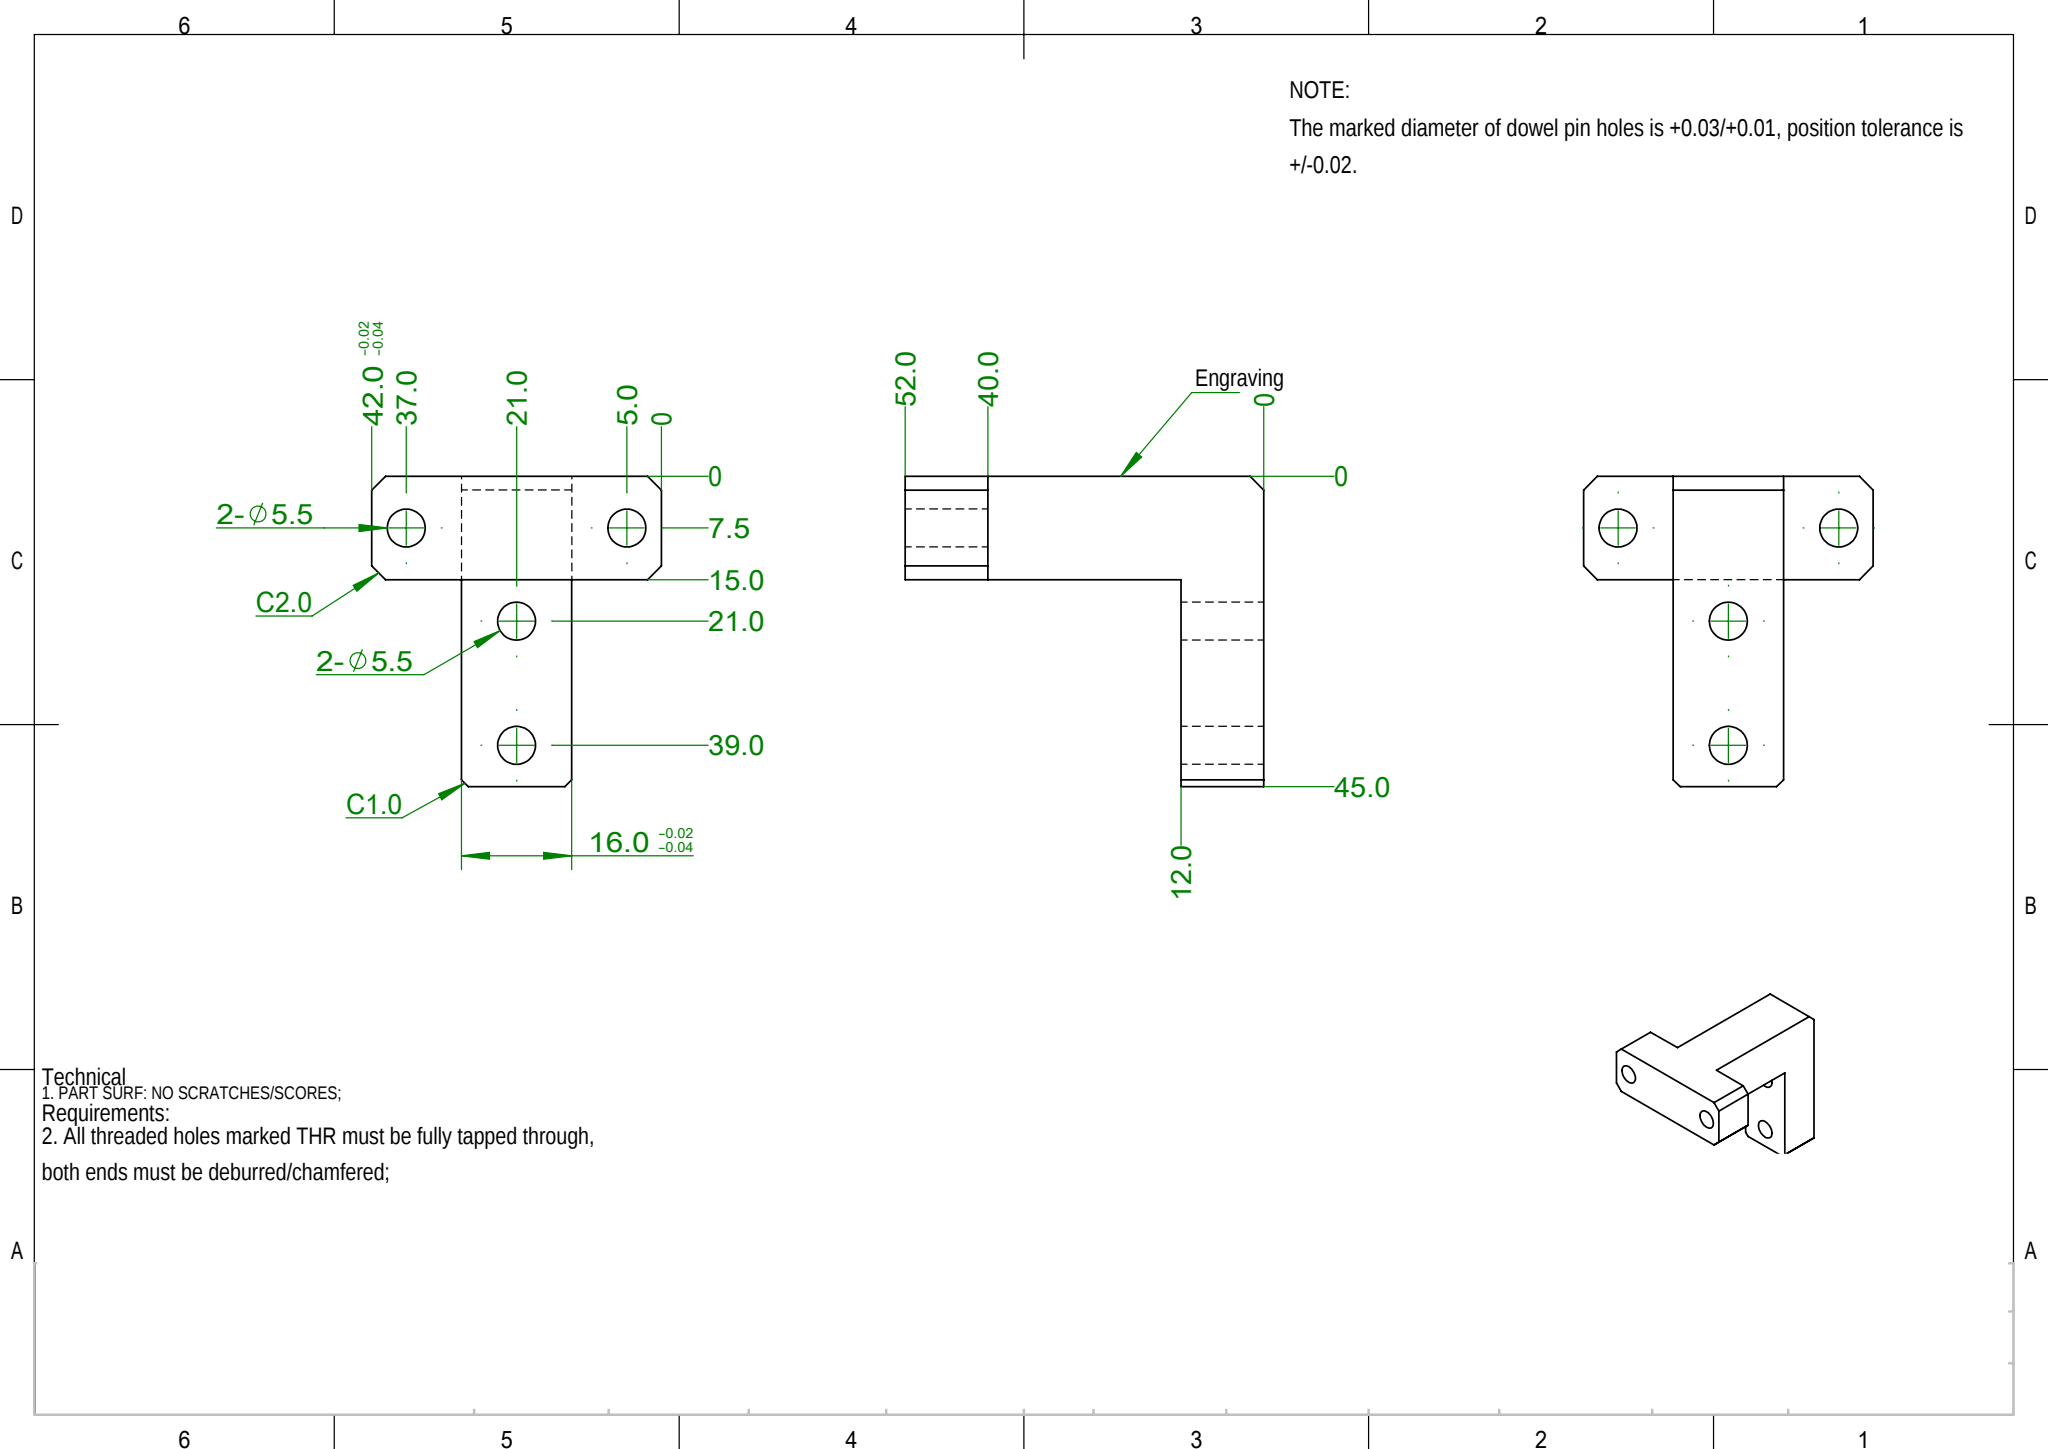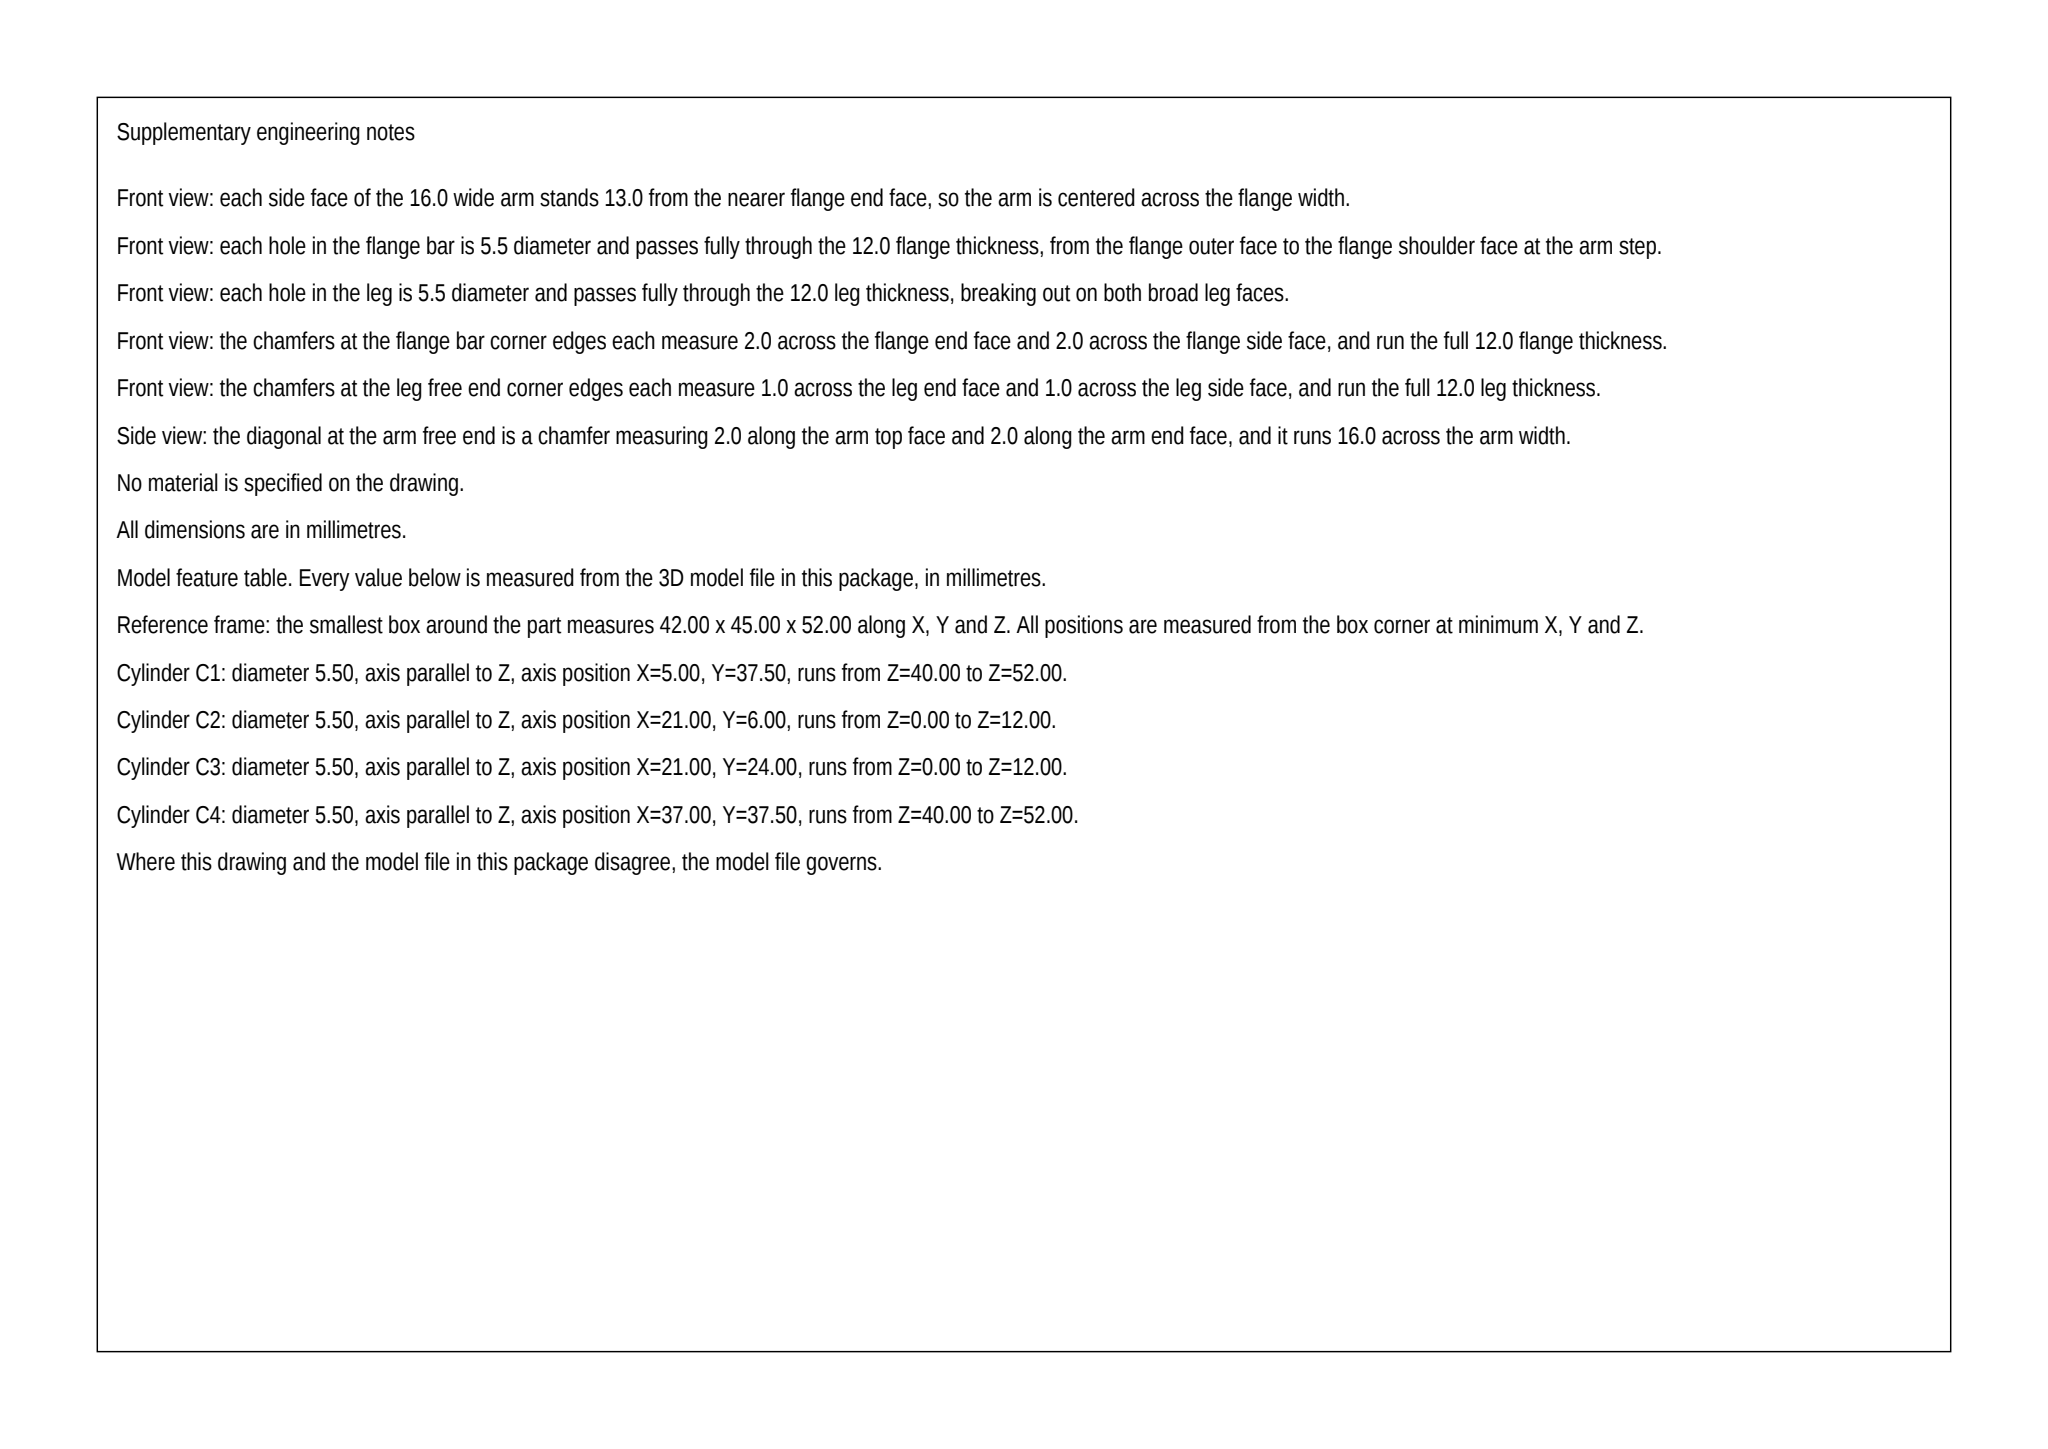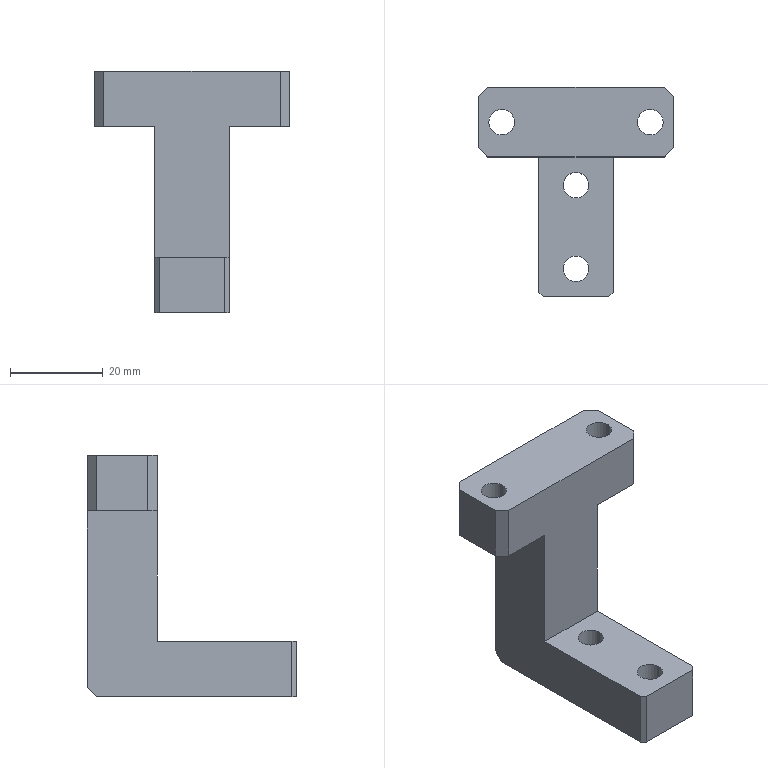Part | SolidWorks | mm | 1 solid | 27 faces | box 42 x 45 x 52 mm | volume 21640 mm3 | plane 19 | cylinder 8 | commonest cylinder face diameters 5.5 x8
Drawing notes:
ALL DIMENSIONS ARE IN MILLIMETERS (mm). | from the solid: STEP model units are mm (bbox_xyz 42.0 x 45.0 x 52.0 mm)
4X PIN HOLE Ø5.5 +0.03/+0.01, TRUE POS ±0.02, THRU 12 | from the solid: cylinders dia 5.5 axis z length 12 at (5.0,37.5),(37.0,37.5),(21.0,24.0),(21.0,6.0); plate thk z 0-12
OVERALL WIDTH 42.0 MM IN X, MEASURED FROM LEFT END FACE (X=0 DATUM) TO RIGHT END FACE. | from the solid: bbox_xyz = [42.0, 45.0, 52.0]; axis_planes x=0.0 and x=42.0
RIGHT-HAND Ø5.5 THRU HOLE (12 DEEP): AXIS AT X=37.0 FROM LEFT END FACE, Y=7.5 FROM TOP FACE (37.5 FROM BOTTOM Y=0 DATUM). | from the solid: cylinders [5.5, z, [37.0, 37.5], 12.0]; bbox Y=45.0
PIN HOLES: 4X Ø5.5 THRU 12 AT X=5.0 AND X=37.0 (Y=37.5 FROM Y=0 DATUM) AND X=21.0 (Y=24.0 AND Y=6.0 FROM Y=0 DATUM). | from the solid: cylinders [5.5,z,[5.0,37.5],12.0], [5.5,z,[37.0,37.5],12.0], [5.5,z,[21.0,24.0],12.0], [5.5,z,[21.0,6.0],12.0]
STEP:
#1=CARTESIAN_POINT('',(-2.75,-13.5,12.));
#2=VERTEX_POINT('',#1);
#3=CARTESIAN_POINT('',(2.75,-13.5,12.));
#4=VERTEX_POINT('',#3);
#5=CARTESIAN_POINT('',(-0.,-13.5,12.));
#6=DIRECTION('',(0.,0.,1.));
#7=DIRECTION('',(1.,0.,0.));
#8=AXIS2_PLACEMENT_3D('',#5,#6,#7);
#9=CIRCLE('',#8,2.75);
#10=EDGE_CURVE('',#2,#4,#9,.T.);
#11=ORIENTED_EDGE('',*,*,#10,.F.);
#12=CARTESIAN_POINT('',(-2.75,-13.5,24.));
#13=VERTEX_POINT('',#12);
#14=CARTESIAN_POINT('',(-2.75,-13.5,-87.));
#15=DIRECTION('',(0.,0.,1.));
#16=VECTOR('',#15,1000.);
#17=LINE('',#14,#16);
#18=EDGE_CURVE('',#2,#13,#17,.T.);
#19=ORIENTED_EDGE('',*,*,#18,.T.);
#20=CARTESIAN_POINT('',(2.75,-13.5,24.));
#21=VERTEX_POINT('',#20);
#22=CARTESIAN_POINT('',(-0.,-13.5,24.));
#23=DIRECTION('',(0.,0.,1.));
#24=DIRECTION('',(1.,0.,0.));
#25=AXIS2_PLACEMENT_3D('',#22,#23,#24);
#26=CIRCLE('',#25,2.75);
#27=EDGE_CURVE('',#13,#21,#26,.T.);
#28=ORIENTED_EDGE('',*,*,#27,.T.);
#29=CARTESIAN_POINT('',(2.75,-13.5,-87.));
#30=DIRECTION('',(0.,0.,1.));
#31=VECTOR('',#30,1000.);
#32=LINE('',#29,#31);
#33=EDGE_CURVE('',#4,#21,#32,.T.);
#34=ORIENTED_EDGE('',*,*,#33,.F.);
#35=EDGE_LOOP('',(#11,#19,#28,#34));
#36=FACE_OUTER_BOUND('',#35,.T.);
#37=CARTESIAN_POINT('',(-0.,-13.5,-87.));
#38=DIRECTION('',(0.,0.,1.));
#39=DIRECTION('',(1.,0.,0.));
#40=AXIS2_PLACEMENT_3D('',#37,#38,#39);
#41=CYLINDRICAL_SURFACE('',#40,2.75);
#42=ADVANCED_FACE('',(#36),#41,.F.);
#43=CARTESIAN_POINT('',(-2.75,-31.5,12.));
#44=VERTEX_POINT('',#43);
#45=CARTESIAN_POINT('',(2.75,-31.5,12.));
#46=VERTEX_POINT('',#45);
#47=CARTESIAN_POINT('',(-0.,-31.5,12.));
#48=DIRECTION('',(0.,0.,1.));
#49=DIRECTION('',(1.,0.,0.));
#50=AXIS2_PLACEMENT_3D('',#47,#48,#49);
#51=CIRCLE('',#50,2.75);
#52=EDGE_CURVE('',#44,#46,#51,.T.);
#53=ORIENTED_EDGE('',*,*,#52,.F.);
#54=CARTESIAN_POINT('',(-2.75,-31.5,24.));
#55=VERTEX_POINT('',#54);
#56=CARTESIAN_POINT('',(-2.75,-31.5,-87.));
#57=DIRECTION('',(0.,0.,1.));
#58=VECTOR('',#57,1000.);
#59=LINE('',#56,#58);
#60=EDGE_CURVE('',#44,#55,#59,.T.);
#61=ORIENTED_EDGE('',*,*,#60,.T.);
#62=CARTESIAN_POINT('',(2.75,-31.5,24.));
#63=VERTEX_POINT('',#62);
#64=CARTESIAN_POINT('',(-0.,-31.5,24.));
#65=DIRECTION('',(0.,0.,1.));
#66=DIRECTION('',(1.,0.,0.));
#67=AXIS2_PLACEMENT_3D('',#64,#65,#66);
#68=CIRCLE('',#67,2.75);
#69=EDGE_CURVE('',#55,#63,#68,.T.);
#70=ORIENTED_EDGE('',*,*,#69,.T.);
#71=CARTESIAN_POINT('',(2.75,-31.5,-87.));
#72=DIRECTION('',(0.,0.,1.));
#73=VECTOR('',#72,1000.);
#74=LINE('',#71,#73);
#75=EDGE_CURVE('',#46,#63,#74,.T.);
#76=ORIENTED_EDGE('',*,*,#75,.F.);
#77=EDGE_LOOP('',(#53,#61,#70,#76));
#78=FACE_OUTER_BOUND('',#77,.T.);
#79=CARTESIAN_POINT('',(-0.,-31.5,-87.));
#80=DIRECTION('',(0.,0.,1.));
#81=DIRECTION('',(1.,0.,0.));
#82=AXIS2_PLACEMENT_3D('',#79,#80,#81);
#83=CYLINDRICAL_SURFACE('',#82,2.75);
#84=ADVANCED_FACE('',(#78),#83,.F.);
#85=CARTESIAN_POINT('',(-18.75,0.,64.));
#86=VERTEX_POINT('',#85);
#87=CARTESIAN_POINT('',(-13.25,0.,64.));
#88=VERTEX_POINT('',#87);
#89=CARTESIAN_POINT('',(-16.,0.,64.));
#90=DIRECTION('',(0.,0.,1.));
#91=DIRECTION('',(-1.,0.,0.));
#92=AXIS2_PLACEMENT_3D('',#89,#90,#91);
#93=CIRCLE('',#92,2.75);
#94=EDGE_CURVE('',#86,#88,#93,.T.);
#95=ORIENTED_EDGE('',*,*,#94,.T.);
#96=CARTESIAN_POINT('',(-13.25,0.,52.));
#97=VERTEX_POINT('',#96);
#98=CARTESIAN_POINT('',(-13.25,0.,111.));
#99=DIRECTION('',(0.,0.,-1.));
#100=VECTOR('',#99,1000.);
#101=LINE('',#98,#100);
#102=EDGE_CURVE('',#88,#97,#101,.T.);
#103=ORIENTED_EDGE('',*,*,#102,.T.);
#104=CARTESIAN_POINT('',(-18.75,0.,52.));
#105=VERTEX_POINT('',#104);
#106=CARTESIAN_POINT('',(-16.,0.,52.));
#107=DIRECTION('',(-0.,0.,-1.));
#108=DIRECTION('',(1.,0.,0.));
#109=AXIS2_PLACEMENT_3D('',#106,#107,#108);
#110=CIRCLE('',#109,2.75);
#111=EDGE_CURVE('',#97,#105,#110,.T.);
#112=ORIENTED_EDGE('',*,*,#111,.T.);
#113=CARTESIAN_POINT('',(-18.75,0.,111.));
#114=DIRECTION('',(0.,0.,-1.));
#115=VECTOR('',#114,1000.);
#116=LINE('',#113,#115);
#117=EDGE_CURVE('',#86,#105,#116,.T.);
#118=ORIENTED_EDGE('',*,*,#117,.F.);
#119=EDGE_LOOP('',(#95,#103,#112,#118));
#120=FACE_OUTER_BOUND('',#119,.T.);
#121=CARTESIAN_POINT('',(-16.,0.,111.));
#122=DIRECTION('',(0.,0.,-1.));
#123=DIRECTION('',(-1.,0.,0.));
#124=AXIS2_PLACEMENT_3D('',#121,#122,#123);
#125=CYLINDRICAL_SURFACE('',#124,2.75);
#126=ADVANCED_FACE('',(#120),#125,.F.);
#127=CARTESIAN_POINT('',(13.25,0.,64.));
#128=VERTEX_POINT('',#127);
#129=CARTESIAN_POINT('',(18.75,0.,64.));
#130=VERTEX_POINT('',#129);
#131=CARTESIAN_POINT('',(16.,0.,64.));
#132=DIRECTION('',(0.,0.,1.));
#133=DIRECTION('',(-1.,0.,0.));
#134=AXIS2_PLACEMENT_3D('',#131,#132,#133);
#135=CIRCLE('',#134,2.75);
#136=EDGE_CURVE('',#128,#130,#135,.T.);
#137=ORIENTED_EDGE('',*,*,#136,.T.);
#138=CARTESIAN_POINT('',(18.75,0.,52.));
#139=VERTEX_POINT('',#138);
#140=CARTESIAN_POINT('',(18.75,0.,111.));
#141=DIRECTION('',(0.,0.,-1.));
#142=VECTOR('',#141,1000.);
#143=LINE('',#140,#142);
#144=EDGE_CURVE('',#130,#139,#143,.T.);
#145=ORIENTED_EDGE('',*,*,#144,.T.);
#146=CARTESIAN_POINT('',(13.25,0.,52.));
#147=VERTEX_POINT('',#146);
#148=CARTESIAN_POINT('',(16.,0.,52.));
#149=DIRECTION('',(0.,0.,-1.));
#150=DIRECTION('',(1.,0.,0.));
#151=AXIS2_PLACEMENT_3D('',#148,#149,#150);
#152=CIRCLE('',#151,2.75);
#153=EDGE_CURVE('',#139,#147,#152,.T.);
#154=ORIENTED_EDGE('',*,*,#153,.T.);
#155=CARTESIAN_POINT('',(13.25,0.,111.));
#156=DIRECTION('',(0.,0.,-1.));
#157=VECTOR('',#156,1000.);
#158=LINE('',#155,#157);
#159=EDGE_CURVE('',#128,#147,#158,.T.);
#160=ORIENTED_EDGE('',*,*,#159,.F.);
#161=EDGE_LOOP('',(#137,#145,#154,#160));
#162=FACE_OUTER_BOUND('',#161,.T.);
#163=CARTESIAN_POINT('',(16.,0.,111.));
#164=DIRECTION('',(0.,0.,-1.));
#165=DIRECTION('',(-1.,0.,0.));
#166=AXIS2_PLACEMENT_3D('',#163,#164,#165);
#167=CYLINDRICAL_SURFACE('',#166,2.75);
#168=ADVANCED_FACE('',(#162),#167,.F.);
#169=CARTESIAN_POINT('',(8.,-7.5,24.));
#170=VERTEX_POINT('',#169);
#171=CARTESIAN_POINT('',(-8.,-7.5,24.));
#172=VERTEX_POINT('',#171);
#173=CARTESIAN_POINT('',(8.,-7.5,24.));
#174=DIRECTION('',(-1.,0.,-0.));
#175=VECTOR('',#174,1000.);
#176=LINE('',#173,#175);
#177=EDGE_CURVE('',#170,#172,#176,.T.);
#178=ORIENTED_EDGE('',*,*,#177,.F.);
#179=CARTESIAN_POINT('',(8.,-7.5,52.));
#180=VERTEX_POINT('',#179);
#181=CARTESIAN_POINT('',(8.,-7.5,0.));
#182=DIRECTION('',(0.,0.,1.));
#183=VECTOR('',#182,1000.);
#184=LINE('',#181,#183);
#185=EDGE_CURVE('',#170,#180,#184,.T.);
#186=ORIENTED_EDGE('',*,*,#185,.T.);
#187=CARTESIAN_POINT('',(19.,-7.5,52.));
#188=VERTEX_POINT('',#187);
#189=CARTESIAN_POINT('',(-0.,-7.5,52.));
#190=DIRECTION('',(1.,0.,0.));
#191=VECTOR('',#190,1000.);
#192=LINE('',#189,#191);
#193=EDGE_CURVE('',#180,#188,#192,.T.);
#194=ORIENTED_EDGE('',*,*,#193,.T.);
#195=CARTESIAN_POINT('',(19.,-7.5,64.));
#196=VERTEX_POINT('',#195);
#197=CARTESIAN_POINT('',(19.,-7.5,0.));
#198=DIRECTION('',(-0.,0.,1.));
#199=VECTOR('',#198,1000.);
#200=LINE('',#197,#199);
#201=EDGE_CURVE('',#188,#196,#200,.T.);
#202=ORIENTED_EDGE('',*,*,#201,.T.);
#203=CARTESIAN_POINT('',(-19.,-7.5,64.));
#204=VERTEX_POINT('',#203);
#205=CARTESIAN_POINT('',(-21.,-7.5,64.));
#206=DIRECTION('',(1.,0.,0.));
#207=VECTOR('',#206,1000.);
#208=LINE('',#205,#207);
#209=EDGE_CURVE('',#204,#196,#208,.T.);
#210=ORIENTED_EDGE('',*,*,#209,.F.);
#211=CARTESIAN_POINT('',(-19.,-7.5,52.));
#212=VERTEX_POINT('',#211);
#213=CARTESIAN_POINT('',(-19.,-7.5,0.));
#214=DIRECTION('',(-0.,0.,-1.));
#215=VECTOR('',#214,1000.);
#216=LINE('',#213,#215);
#217=EDGE_CURVE('',#204,#212,#216,.T.);
#218=ORIENTED_EDGE('',*,*,#217,.T.);
#219=CARTESIAN_POINT('',(-8.,-7.5,52.));
#220=VERTEX_POINT('',#219);
#221=CARTESIAN_POINT('',(0.,-7.5,52.));
#222=DIRECTION('',(1.,0.,-0.));
#223=VECTOR('',#222,1000.);
#224=LINE('',#221,#223);
#225=EDGE_CURVE('',#212,#220,#224,.T.);
#226=ORIENTED_EDGE('',*,*,#225,.T.);
#227=CARTESIAN_POINT('',(-8.,-7.5,0.));
#228=DIRECTION('',(0.,0.,-1.));
#229=VECTOR('',#228,1000.);
#230=LINE('',#227,#229);
#231=EDGE_CURVE('',#220,#172,#230,.T.);
#232=ORIENTED_EDGE('',*,*,#231,.T.);
#233=EDGE_LOOP('',(#178,#186,#194,#202,#210,#218,#226,#232));
#234=FACE_OUTER_BOUND('',#233,.T.);
#235=CARTESIAN_POINT('',(0.,-7.5,0.));
#236=DIRECTION('',(0.,1.,0.));
#237=DIRECTION('',(0.,0.,1.));
#238=AXIS2_PLACEMENT_3D('',#235,#236,#237);
#239=PLANE('',#238);
#240=ADVANCED_FACE('',(#234),#239,.F.);
#241=CARTESIAN_POINT('',(-21.,5.5,52.));
#242=VERTEX_POINT('',#241);
#243=CARTESIAN_POINT('',(-21.,-5.5,52.));
#244=VERTEX_POINT('',#243);
#245=CARTESIAN_POINT('',(-21.,7.5,52.));
#246=DIRECTION('',(0.,-1.,0.));
#247=VECTOR('',#246,1000.);
#248=LINE('',#245,#247);
#249=EDGE_CURVE('',#242,#244,#248,.T.);
#250=ORIENTED_EDGE('',*,*,#249,.T.);
#251=CARTESIAN_POINT('',(-21.,-5.5,64.));
#252=VERTEX_POINT('',#251);
#253=CARTESIAN_POINT('',(-21.,-5.5,0.));
#254=DIRECTION('',(0.,0.,1.));
#255=VECTOR('',#254,1000.);
#256=LINE('',#253,#255);
#257=EDGE_CURVE('',#244,#252,#256,.T.);
#258=ORIENTED_EDGE('',*,*,#257,.T.);
#259=CARTESIAN_POINT('',(-21.,5.5,64.));
#260=VERTEX_POINT('',#259);
#261=CARTESIAN_POINT('',(-21.,7.5,64.));
#262=DIRECTION('',(0.,-1.,0.));
#263=VECTOR('',#262,1000.);
#264=LINE('',#261,#263);
#265=EDGE_CURVE('',#260,#252,#264,.T.);
#266=ORIENTED_EDGE('',*,*,#265,.F.);
#267=CARTESIAN_POINT('',(-21.,5.5,52.));
#268=DIRECTION('',(-0.,0.,-1.));
#269=VECTOR('',#268,1000.);
#270=LINE('',#267,#269);
#271=EDGE_CURVE('',#260,#242,#270,.T.);
#272=ORIENTED_EDGE('',*,*,#271,.T.);
#273=EDGE_LOOP('',(#250,#258,#266,#272));
#274=FACE_OUTER_BOUND('',#273,.T.);
#275=CARTESIAN_POINT('',(-21.,7.5,0.));
#276=DIRECTION('',(1.,0.,-0.));
#277=DIRECTION('',(-0.,0.,-1.));
#278=AXIS2_PLACEMENT_3D('',#275,#276,#277);
#279=PLANE('',#278);
#280=ADVANCED_FACE('',(#274),#279,.F.);
#281=CARTESIAN_POINT('',(21.,5.5,64.));
#282=VERTEX_POINT('',#281);
#283=CARTESIAN_POINT('',(21.,-5.5,64.));
#284=VERTEX_POINT('',#283);
#285=CARTESIAN_POINT('',(21.,7.5,64.));
#286=DIRECTION('',(0.,-1.,0.));
#287=VECTOR('',#286,1000.);
#288=LINE('',#285,#287);
#289=EDGE_CURVE('',#282,#284,#288,.T.);
#290=ORIENTED_EDGE('',*,*,#289,.T.);
#291=CARTESIAN_POINT('',(21.,-5.5,52.));
#292=VERTEX_POINT('',#291);
#293=CARTESIAN_POINT('',(21.,-5.5,0.));
#294=DIRECTION('',(0.,0.,-1.));
#295=VECTOR('',#294,1000.);
#296=LINE('',#293,#295);
#297=EDGE_CURVE('',#284,#292,#296,.T.);
#298=ORIENTED_EDGE('',*,*,#297,.T.);
#299=CARTESIAN_POINT('',(21.,5.5,52.));
#300=VERTEX_POINT('',#299);
#301=CARTESIAN_POINT('',(21.,7.5,52.));
#302=DIRECTION('',(0.,1.,0.));
#303=VECTOR('',#302,1000.);
#304=LINE('',#301,#303);
#305=EDGE_CURVE('',#292,#300,#304,.T.);
#306=ORIENTED_EDGE('',*,*,#305,.T.);
#307=CARTESIAN_POINT('',(21.,5.5,64.));
#308=DIRECTION('',(-0.,0.,1.));
#309=VECTOR('',#308,1000.);
#310=LINE('',#307,#309);
#311=EDGE_CURVE('',#300,#282,#310,.T.);
#312=ORIENTED_EDGE('',*,*,#311,.T.);
#313=EDGE_LOOP('',(#290,#298,#306,#312));
#314=FACE_OUTER_BOUND('',#313,.T.);
#315=CARTESIAN_POINT('',(21.,7.5,0.));
#316=DIRECTION('',(-1.,0.,-0.));
#317=DIRECTION('',(-0.,0.,1.));
#318=AXIS2_PLACEMENT_3D('',#315,#316,#317);
#319=PLANE('',#318);
#320=ADVANCED_FACE('',(#314),#319,.F.);
#321=ORIENTED_EDGE('',*,*,#94,.F.);
#322=CARTESIAN_POINT('',(-16.,0.,64.));
#323=DIRECTION('',(0.,0.,1.));
#324=DIRECTION('',(-1.,0.,0.));
#325=AXIS2_PLACEMENT_3D('',#322,#323,#324);
#326=CIRCLE('',#325,2.75);
#327=EDGE_CURVE('',#88,#86,#326,.T.);
#328=ORIENTED_EDGE('',*,*,#327,.F.);
#329=EDGE_LOOP('',(#321,#328));
#330=FACE_BOUND('',#329,.T.);
#331=ORIENTED_EDGE('',*,*,#136,.F.);
#332=CARTESIAN_POINT('',(16.,0.,64.));
#333=DIRECTION('',(0.,0.,1.));
#334=DIRECTION('',(-1.,0.,0.));
#335=AXIS2_PLACEMENT_3D('',#332,#333,#334);
#336=CIRCLE('',#335,2.75);
#337=EDGE_CURVE('',#130,#128,#336,.T.);
#338=ORIENTED_EDGE('',*,*,#337,.F.);
#339=EDGE_LOOP('',(#331,#338));
#340=FACE_BOUND('',#339,.T.);
#341=ORIENTED_EDGE('',*,*,#265,.T.);
#342=CARTESIAN_POINT('',(-21.,-5.5,64.));
#343=DIRECTION('',(0.7071,-0.7071,0.));
#344=VECTOR('',#343,1000.);
#345=LINE('',#342,#344);
#346=EDGE_CURVE('',#252,#204,#345,.T.);
#347=ORIENTED_EDGE('',*,*,#346,.T.);
#348=ORIENTED_EDGE('',*,*,#209,.T.);
#349=CARTESIAN_POINT('',(21.,-5.5,64.));
#350=DIRECTION('',(0.7071,0.7071,0.));
#351=VECTOR('',#350,1000.);
#352=LINE('',#349,#351);
#353=EDGE_CURVE('',#196,#284,#352,.T.);
#354=ORIENTED_EDGE('',*,*,#353,.T.);
#355=ORIENTED_EDGE('',*,*,#289,.F.);
#356=CARTESIAN_POINT('',(19.,7.5,64.));
#357=VERTEX_POINT('',#356);
#358=CARTESIAN_POINT('',(19.,7.5,64.));
#359=DIRECTION('',(-0.7071,0.7071,0.));
#360=VECTOR('',#359,1000.);
#361=LINE('',#358,#360);
#362=EDGE_CURVE('',#282,#357,#361,.T.);
#363=ORIENTED_EDGE('',*,*,#362,.T.);
#364=CARTESIAN_POINT('',(-19.,7.5,64.));
#365=VERTEX_POINT('',#364);
#366=CARTESIAN_POINT('',(-21.,7.5,64.));
#367=DIRECTION('',(1.,0.,0.));
#368=VECTOR('',#367,1000.);
#369=LINE('',#366,#368);
#370=EDGE_CURVE('',#365,#357,#369,.T.);
#371=ORIENTED_EDGE('',*,*,#370,.F.);
#372=CARTESIAN_POINT('',(-19.,7.5,64.));
#373=DIRECTION('',(-0.7071,-0.7071,0.));
#374=VECTOR('',#373,1000.);
#375=LINE('',#372,#374);
#376=EDGE_CURVE('',#365,#260,#375,.T.);
#377=ORIENTED_EDGE('',*,*,#376,.T.);
#378=EDGE_LOOP('',(#341,#347,#348,#354,#355,#363,#371,#377));
#379=FACE_OUTER_BOUND('',#378,.T.);
#380=CARTESIAN_POINT('',(-21.,7.5,64.));
#381=DIRECTION('',(0.,0.,-1.));
#382=DIRECTION('',(-1.,0.,0.));
#383=AXIS2_PLACEMENT_3D('',#380,#381,#382);
#384=PLANE('',#383);
#385=ADVANCED_FACE('',(#330,#340,#379),#384,.F.);
#386=CARTESIAN_POINT('',(-0.,-13.5,12.));
#387=DIRECTION('',(0.,0.,1.));
#388=DIRECTION('',(1.,0.,0.));
#389=AXIS2_PLACEMENT_3D('',#386,#387,#388);
#390=CIRCLE('',#389,2.75);
#391=EDGE_CURVE('',#4,#2,#390,.T.);
#392=ORIENTED_EDGE('',*,*,#391,.T.);
#393=ORIENTED_EDGE('',*,*,#10,.T.);
#394=EDGE_LOOP('',(#392,#393));
#395=FACE_BOUND('',#394,.T.);
#396=CARTESIAN_POINT('',(-0.,-31.5,12.));
#397=DIRECTION('',(0.,0.,1.));
#398=DIRECTION('',(1.,0.,0.));
#399=AXIS2_PLACEMENT_3D('',#396,#397,#398);
#400=CIRCLE('',#399,2.75);
#401=EDGE_CURVE('',#46,#44,#400,.T.);
#402=ORIENTED_EDGE('',*,*,#401,.T.);
#403=ORIENTED_EDGE('',*,*,#52,.T.);
#404=EDGE_LOOP('',(#402,#403));
#405=FACE_BOUND('',#404,.T.);
#406=CARTESIAN_POINT('',(-8.,-36.5,12.));
#407=VERTEX_POINT('',#406);
#408=CARTESIAN_POINT('',(-8.,5.5,12.));
#409=VERTEX_POINT('',#408);
#410=CARTESIAN_POINT('',(-8.,7.5,12.));
#411=DIRECTION('',(0.,1.,0.));
#412=VECTOR('',#411,1000.);
#413=LINE('',#410,#412);
#414=EDGE_CURVE('',#407,#409,#413,.T.);
#415=ORIENTED_EDGE('',*,*,#414,.T.);
#416=CARTESIAN_POINT('',(8.,5.5,12.));
#417=VERTEX_POINT('',#416);
#418=CARTESIAN_POINT('',(8.,5.5,12.));
#419=DIRECTION('',(1.,0.,0.));
#420=VECTOR('',#419,1000.);
#421=LINE('',#418,#420);
#422=EDGE_CURVE('',#409,#417,#421,.T.);
#423=ORIENTED_EDGE('',*,*,#422,.T.);
#424=CARTESIAN_POINT('',(8.,-36.5,12.));
#425=VERTEX_POINT('',#424);
#426=CARTESIAN_POINT('',(8.,7.5,12.));
#427=DIRECTION('',(0.,-1.,0.));
#428=VECTOR('',#427,1000.);
#429=LINE('',#426,#428);
#430=EDGE_CURVE('',#417,#425,#429,.T.);
#431=ORIENTED_EDGE('',*,*,#430,.T.);
#432=CARTESIAN_POINT('',(7.,-37.5,12.));
#433=VERTEX_POINT('',#432);
#434=CARTESIAN_POINT('',(7.,-37.5,12.));
#435=DIRECTION('',(-0.7071,-0.7071,0.));
#436=VECTOR('',#435,1000.);
#437=LINE('',#434,#436);
#438=EDGE_CURVE('',#425,#433,#437,.T.);
#439=ORIENTED_EDGE('',*,*,#438,.T.);
#440=CARTESIAN_POINT('',(-7.,-37.5,12.));
#441=VERTEX_POINT('',#440);
#442=CARTESIAN_POINT('',(8.,-37.5,12.));
#443=DIRECTION('',(1.,0.,0.));
#444=VECTOR('',#443,1000.);
#445=LINE('',#442,#444);
#446=EDGE_CURVE('',#441,#433,#445,.T.);
#447=ORIENTED_EDGE('',*,*,#446,.F.);
#448=CARTESIAN_POINT('',(-7.,-37.5,12.));
#449=DIRECTION('',(-0.7071,0.7071,0.));
#450=VECTOR('',#449,1000.);
#451=LINE('',#448,#450);
#452=EDGE_CURVE('',#441,#407,#451,.T.);
#453=ORIENTED_EDGE('',*,*,#452,.T.);
#454=EDGE_LOOP('',(#415,#423,#431,#439,#447,#453));
#455=FACE_OUTER_BOUND('',#454,.T.);
#456=CARTESIAN_POINT('',(-21.,7.5,12.));
#457=DIRECTION('',(0.,0.,1.));
#458=DIRECTION('',(1.,0.,0.));
#459=AXIS2_PLACEMENT_3D('',#456,#457,#458);
#460=PLANE('',#459);
#461=ADVANCED_FACE('',(#395,#405,#455),#460,.F.);
#462=CARTESIAN_POINT('',(8.,7.5,14.));
#463=VERTEX_POINT('',#462);
#464=CARTESIAN_POINT('',(8.,7.5,52.));
#465=VERTEX_POINT('',#464);
#466=CARTESIAN_POINT('',(8.,7.5,52.));
#467=DIRECTION('',(0.,0.,1.));
#468=VECTOR('',#467,1000.);
#469=LINE('',#466,#468);
#470=EDGE_CURVE('',#463,#465,#469,.T.);
#471=ORIENTED_EDGE('',*,*,#470,.F.);
#472=CARTESIAN_POINT('',(-8.,7.5,14.));
#473=VERTEX_POINT('',#472);
#474=CARTESIAN_POINT('',(-8.,7.5,14.));
#475=DIRECTION('',(-1.,0.,0.));
#476=VECTOR('',#475,1000.);
#477=LINE('',#474,#476);
#478=EDGE_CURVE('',#463,#473,#477,.T.);
#479=ORIENTED_EDGE('',*,*,#478,.T.);
#480=CARTESIAN_POINT('',(-8.,7.5,52.));
#481=VERTEX_POINT('',#480);
#482=CARTESIAN_POINT('',(-8.,7.5,52.));
#483=DIRECTION('',(0.,0.,-1.));
#484=VECTOR('',#483,1000.);
#485=LINE('',#482,#484);
#486=EDGE_CURVE('',#481,#473,#485,.T.);
#487=ORIENTED_EDGE('',*,*,#486,.F.);
#488=CARTESIAN_POINT('',(-19.,7.5,52.));
#489=VERTEX_POINT('',#488);
#490=CARTESIAN_POINT('',(-28.,7.5,52.));
#491=DIRECTION('',(1.,0.,-0.));
#492=VECTOR('',#491,1000.);
#493=LINE('',#490,#492);
#494=EDGE_CURVE('',#489,#481,#493,.T.);
#495=ORIENTED_EDGE('',*,*,#494,.F.);
#496=CARTESIAN_POINT('',(-19.,7.5,64.));
#497=DIRECTION('',(0.,0.,1.));
#498=VECTOR('',#497,1000.);
#499=LINE('',#496,#498);
#500=EDGE_CURVE('',#489,#365,#499,.T.);
#501=ORIENTED_EDGE('',*,*,#500,.T.);
#502=ORIENTED_EDGE('',*,*,#370,.T.);
#503=CARTESIAN_POINT('',(19.,7.5,52.));
#504=VERTEX_POINT('',#503);
#505=CARTESIAN_POINT('',(19.,7.5,52.));
#506=DIRECTION('',(0.,0.,-1.));
#507=VECTOR('',#506,1000.);
#508=LINE('',#505,#507);
#509=EDGE_CURVE('',#357,#504,#508,.T.);
#510=ORIENTED_EDGE('',*,*,#509,.T.);
#511=CARTESIAN_POINT('',(28.,7.5,52.));
#512=DIRECTION('',(1.,0.,0.));
#513=VECTOR('',#512,1000.);
#514=LINE('',#511,#513);
#515=EDGE_CURVE('',#465,#504,#514,.T.);
#516=ORIENTED_EDGE('',*,*,#515,.F.);
#517=EDGE_LOOP('',(#471,#479,#487,#495,#501,#502,#510,#516));
#518=FACE_OUTER_BOUND('',#517,.T.);
#519=CARTESIAN_POINT('',(0.,7.5,0.));
#520=DIRECTION('',(0.,1.,0.));
#521=DIRECTION('',(0.,0.,1.));
#522=AXIS2_PLACEMENT_3D('',#519,#520,#521);
#523=PLANE('',#522);
#524=ADVANCED_FACE('',(#518),#523,.T.);
#525=CARTESIAN_POINT('',(16.,0.,52.));
#526=DIRECTION('',(0.,0.,-1.));
#527=DIRECTION('',(1.,0.,0.));
#528=AXIS2_PLACEMENT_3D('',#525,#526,#527);
#529=CIRCLE('',#528,2.75);
#530=EDGE_CURVE('',#147,#139,#529,.T.);
#531=ORIENTED_EDGE('',*,*,#530,.F.);
#532=ORIENTED_EDGE('',*,*,#153,.F.);
#533=EDGE_LOOP('',(#531,#532));
#534=FACE_BOUND('',#533,.T.);
#535=ORIENTED_EDGE('',*,*,#305,.F.);
#536=CARTESIAN_POINT('',(21.,-5.5,52.));
#537=DIRECTION('',(-0.7071,-0.7071,-0.));
#538=VECTOR('',#537,1000.);
#539=LINE('',#536,#538);
#540=EDGE_CURVE('',#292,#188,#539,.T.);
#541=ORIENTED_EDGE('',*,*,#540,.T.);
#542=ORIENTED_EDGE('',*,*,#193,.F.);
#543=CARTESIAN_POINT('',(8.,-103.5,52.));
#544=DIRECTION('',(0.,1.,0.));
#545=VECTOR('',#544,1000.);
#546=LINE('',#543,#545);
#547=EDGE_CURVE('',#180,#465,#546,.T.);
#548=ORIENTED_EDGE('',*,*,#547,.T.);
#549=ORIENTED_EDGE('',*,*,#515,.T.);
#550=CARTESIAN_POINT('',(19.,7.5,52.));
#551=DIRECTION('',(0.7071,-0.7071,0.));
#552=VECTOR('',#551,1000.);
#553=LINE('',#550,#552);
#554=EDGE_CURVE('',#504,#300,#553,.T.);
#555=ORIENTED_EDGE('',*,*,#554,.T.);
#556=EDGE_LOOP('',(#535,#541,#542,#548,#549,#555));
#557=FACE_OUTER_BOUND('',#556,.T.);
#558=CARTESIAN_POINT('',(28.,-103.5,52.));
#559=DIRECTION('',(-0.,0.,1.));
#560=DIRECTION('',(1.,0.,0.));
#561=AXIS2_PLACEMENT_3D('',#558,#559,#560);
#562=PLANE('',#561);
#563=ADVANCED_FACE('',(#534,#557),#562,.F.);
#564=ORIENTED_EDGE('',*,*,#430,.F.);
#565=CARTESIAN_POINT('',(8.,7.5,14.));
#566=DIRECTION('',(0.,0.7071,0.7071));
#567=VECTOR('',#566,1000.);
#568=LINE('',#565,#567);
#569=EDGE_CURVE('',#417,#463,#568,.T.);
#570=ORIENTED_EDGE('',*,*,#569,.T.);
#571=ORIENTED_EDGE('',*,*,#470,.T.);
#572=ORIENTED_EDGE('',*,*,#547,.F.);
#573=ORIENTED_EDGE('',*,*,#185,.F.);
#574=CARTESIAN_POINT('',(8.,-36.5,24.));
#575=VERTEX_POINT('',#574);
#576=CARTESIAN_POINT('',(8.,-37.5,24.));
#577=DIRECTION('',(0.,1.,0.));
#578=VECTOR('',#577,1000.);
#579=LINE('',#576,#578);
#580=EDGE_CURVE('',#575,#170,#579,.T.);
#581=ORIENTED_EDGE('',*,*,#580,.F.);
#582=CARTESIAN_POINT('',(8.,-36.5,12.));
#583=DIRECTION('',(0.,0.,-1.));
#584=VECTOR('',#583,1000.);
#585=LINE('',#582,#584);
#586=EDGE_CURVE('',#575,#425,#585,.T.);
#587=ORIENTED_EDGE('',*,*,#586,.T.);
#588=EDGE_LOOP('',(#564,#570,#571,#572,#573,#581,#587));
#589=FACE_OUTER_BOUND('',#588,.T.);
#590=CARTESIAN_POINT('',(8.,-103.5,52.));
#591=DIRECTION('',(-1.,0.,0.));
#592=DIRECTION('',(0.,0.,1.));
#593=AXIS2_PLACEMENT_3D('',#590,#591,#592);
#594=PLANE('',#593);
#595=ADVANCED_FACE('',(#589),#594,.F.);
#596=CARTESIAN_POINT('',(-16.,0.,52.));
#597=DIRECTION('',(-0.,0.,-1.));
#598=DIRECTION('',(1.,0.,0.));
#599=AXIS2_PLACEMENT_3D('',#596,#597,#598);
#600=CIRCLE('',#599,2.75);
#601=EDGE_CURVE('',#105,#97,#600,.T.);
#602=ORIENTED_EDGE('',*,*,#601,.F.);
#603=ORIENTED_EDGE('',*,*,#111,.F.);
#604=EDGE_LOOP('',(#602,#603));
#605=FACE_BOUND('',#604,.T.);
#606=ORIENTED_EDGE('',*,*,#225,.F.);
#607=CARTESIAN_POINT('',(-21.,-5.5,52.));
#608=DIRECTION('',(-0.7071,0.7071,0.));
#609=VECTOR('',#608,1000.);
#610=LINE('',#607,#609);
#611=EDGE_CURVE('',#212,#244,#610,.T.);
#612=ORIENTED_EDGE('',*,*,#611,.T.);
#613=ORIENTED_EDGE('',*,*,#249,.F.);
#614=CARTESIAN_POINT('',(-19.,7.5,52.));
#615=DIRECTION('',(0.7071,0.7071,-0.));
#616=VECTOR('',#615,1000.);
#617=LINE('',#614,#616);
#618=EDGE_CURVE('',#242,#489,#617,.T.);
#619=ORIENTED_EDGE('',*,*,#618,.T.);
#620=ORIENTED_EDGE('',*,*,#494,.T.);
#621=CARTESIAN_POINT('',(-8.,-103.5,52.));
#622=DIRECTION('',(0.,1.,0.));
#623=VECTOR('',#622,1000.);
#624=LINE('',#621,#623);
#625=EDGE_CURVE('',#220,#481,#624,.T.);
#626=ORIENTED_EDGE('',*,*,#625,.F.);
#627=EDGE_LOOP('',(#606,#612,#613,#619,#620,#626));
#628=FACE_OUTER_BOUND('',#627,.T.);
#629=CARTESIAN_POINT('',(-28.,-103.5,52.));
#630=DIRECTION('',(0.,0.,1.));
#631=DIRECTION('',(1.,0.,-0.));
#632=AXIS2_PLACEMENT_3D('',#629,#630,#631);
#633=PLANE('',#632);
#634=ADVANCED_FACE('',(#605,#628),#633,.F.);
#635=ORIENTED_EDGE('',*,*,#486,.T.);
#636=CARTESIAN_POINT('',(-8.,7.5,14.));
#637=DIRECTION('',(0.,-0.7071,-0.7071));
#638=VECTOR('',#637,1000.);
#639=LINE('',#636,#638);
#640=EDGE_CURVE('',#473,#409,#639,.T.);
#641=ORIENTED_EDGE('',*,*,#640,.T.);
#642=ORIENTED_EDGE('',*,*,#414,.F.);
#643=CARTESIAN_POINT('',(-8.,-36.5,24.));
#644=VERTEX_POINT('',#643);
#645=CARTESIAN_POINT('',(-8.,-36.5,24.));
#646=DIRECTION('',(0.,0.,1.));
#647=VECTOR('',#646,1000.);
#648=LINE('',#645,#647);
#649=EDGE_CURVE('',#407,#644,#648,.T.);
#650=ORIENTED_EDGE('',*,*,#649,.T.);
#651=CARTESIAN_POINT('',(-8.,-37.5,24.));
#652=DIRECTION('',(0.,1.,0.));
#653=VECTOR('',#652,1000.);
#654=LINE('',#651,#653);
#655=EDGE_CURVE('',#644,#172,#654,.T.);
#656=ORIENTED_EDGE('',*,*,#655,.T.);
#657=ORIENTED_EDGE('',*,*,#231,.F.);
#658=ORIENTED_EDGE('',*,*,#625,.T.);
#659=EDGE_LOOP('',(#635,#641,#642,#650,#656,#657,#658));
#660=FACE_OUTER_BOUND('',#659,.T.);
#661=CARTESIAN_POINT('',(-8.,-103.5,52.));
#662=DIRECTION('',(1.,0.,0.));
#663=DIRECTION('',(0.,0.,-1.));
#664=AXIS2_PLACEMENT_3D('',#661,#662,#663);
#665=PLANE('',#664);
#666=ADVANCED_FACE('',(#660),#665,.F.);
#667=ORIENTED_EDGE('',*,*,#144,.F.);
#668=ORIENTED_EDGE('',*,*,#337,.T.);
#669=ORIENTED_EDGE('',*,*,#159,.T.);
#670=ORIENTED_EDGE('',*,*,#530,.T.);
#671=EDGE_LOOP('',(#667,#668,#669,#670));
#672=FACE_OUTER_BOUND('',#671,.T.);
#673=CARTESIAN_POINT('',(16.,0.,111.));
#674=DIRECTION('',(0.,0.,-1.));
#675=DIRECTION('',(-1.,0.,0.));
#676=AXIS2_PLACEMENT_3D('',#673,#674,#675);
#677=CYLINDRICAL_SURFACE('',#676,2.75);
#678=ADVANCED_FACE('',(#672),#677,.F.);
#679=ORIENTED_EDGE('',*,*,#102,.F.);
#680=ORIENTED_EDGE('',*,*,#327,.T.);
#681=ORIENTED_EDGE('',*,*,#117,.T.);
#682=ORIENTED_EDGE('',*,*,#601,.T.);
#683=EDGE_LOOP('',(#679,#680,#681,#682));
#684=FACE_OUTER_BOUND('',#683,.T.);
#685=CARTESIAN_POINT('',(-16.,0.,111.));
#686=DIRECTION('',(0.,0.,-1.));
#687=DIRECTION('',(-1.,0.,0.));
#688=AXIS2_PLACEMENT_3D('',#685,#686,#687);
#689=CYLINDRICAL_SURFACE('',#688,2.75);
#690=ADVANCED_FACE('',(#684),#689,.F.);
#691=ORIENTED_EDGE('',*,*,#611,.F.);
#692=ORIENTED_EDGE('',*,*,#217,.F.);
#693=ORIENTED_EDGE('',*,*,#346,.F.);
#694=ORIENTED_EDGE('',*,*,#257,.F.);
#695=EDGE_LOOP('',(#691,#692,#693,#694));
#696=FACE_OUTER_BOUND('',#695,.T.);
#697=CARTESIAN_POINT('',(-21.,-5.5,0.));
#698=DIRECTION('',(0.7071,0.7071,-0.));
#699=DIRECTION('',(0.,0.,1.));
#700=AXIS2_PLACEMENT_3D('',#697,#698,#699);
#701=PLANE('',#700);
#702=ADVANCED_FACE('',(#696),#701,.F.);
#703=ORIENTED_EDGE('',*,*,#618,.F.);
#704=ORIENTED_EDGE('',*,*,#271,.F.);
#705=ORIENTED_EDGE('',*,*,#376,.F.);
#706=ORIENTED_EDGE('',*,*,#500,.F.);
#707=EDGE_LOOP('',(#703,#704,#705,#706));
#708=FACE_OUTER_BOUND('',#707,.T.);
#709=CARTESIAN_POINT('',(-19.,7.5,0.));
#710=DIRECTION('',(-0.7071,0.7071,0.));
#711=DIRECTION('',(-0.,0.,-1.));
#712=AXIS2_PLACEMENT_3D('',#709,#710,#711);
#713=PLANE('',#712);
#714=ADVANCED_FACE('',(#708),#713,.T.);
#715=ORIENTED_EDGE('',*,*,#353,.F.);
#716=ORIENTED_EDGE('',*,*,#201,.F.);
#717=ORIENTED_EDGE('',*,*,#540,.F.);
#718=ORIENTED_EDGE('',*,*,#297,.F.);
#719=EDGE_LOOP('',(#715,#716,#717,#718));
#720=FACE_OUTER_BOUND('',#719,.T.);
#721=CARTESIAN_POINT('',(21.,-5.5,0.));
#722=DIRECTION('',(-0.7071,0.7071,-0.));
#723=DIRECTION('',(0.,0.,-1.));
#724=AXIS2_PLACEMENT_3D('',#721,#722,#723);
#725=PLANE('',#724);
#726=ADVANCED_FACE('',(#720),#725,.F.);
#727=ORIENTED_EDGE('',*,*,#362,.F.);
#728=ORIENTED_EDGE('',*,*,#311,.F.);
#729=ORIENTED_EDGE('',*,*,#554,.F.);
#730=ORIENTED_EDGE('',*,*,#509,.F.);
#731=EDGE_LOOP('',(#727,#728,#729,#730));
#732=FACE_OUTER_BOUND('',#731,.T.);
#733=CARTESIAN_POINT('',(19.,7.5,0.));
#734=DIRECTION('',(0.7071,0.7071,0.));
#735=DIRECTION('',(-0.,0.,1.));
#736=AXIS2_PLACEMENT_3D('',#733,#734,#735);
#737=PLANE('',#736);
#738=ADVANCED_FACE('',(#732),#737,.T.);
#739=CARTESIAN_POINT('',(-0.,-13.5,24.));
#740=DIRECTION('',(0.,0.,1.));
#741=DIRECTION('',(1.,0.,0.));
#742=AXIS2_PLACEMENT_3D('',#739,#740,#741);
#743=CIRCLE('',#742,2.75);
#744=EDGE_CURVE('',#21,#13,#743,.T.);
#745=ORIENTED_EDGE('',*,*,#744,.F.);
#746=ORIENTED_EDGE('',*,*,#27,.F.);
#747=EDGE_LOOP('',(#745,#746));
#748=FACE_BOUND('',#747,.T.);
#749=CARTESIAN_POINT('',(-0.,-31.5,24.));
#750=DIRECTION('',(0.,0.,1.));
#751=DIRECTION('',(1.,0.,0.));
#752=AXIS2_PLACEMENT_3D('',#749,#750,#751);
#753=CIRCLE('',#752,2.75);
#754=EDGE_CURVE('',#63,#55,#753,.T.);
#755=ORIENTED_EDGE('',*,*,#754,.F.);
#756=ORIENTED_EDGE('',*,*,#69,.F.);
#757=EDGE_LOOP('',(#755,#756));
#758=FACE_BOUND('',#757,.T.);
#759=CARTESIAN_POINT('',(7.,-37.5,24.));
#760=VERTEX_POINT('',#759);
#761=CARTESIAN_POINT('',(-7.,-37.5,24.));
#762=VERTEX_POINT('',#761);
#763=CARTESIAN_POINT('',(8.,-37.5,24.));
#764=DIRECTION('',(-1.,0.,-0.));
#765=VECTOR('',#764,1000.);
#766=LINE('',#763,#765);
#767=EDGE_CURVE('',#760,#762,#766,.T.);
#768=ORIENTED_EDGE('',*,*,#767,.F.);
#769=CARTESIAN_POINT('',(7.,-37.5,24.));
#770=DIRECTION('',(0.7071,0.7071,0.));
#771=VECTOR('',#770,1000.);
#772=LINE('',#769,#771);
#773=EDGE_CURVE('',#760,#575,#772,.T.);
#774=ORIENTED_EDGE('',*,*,#773,.T.);
#775=ORIENTED_EDGE('',*,*,#580,.T.);
#776=ORIENTED_EDGE('',*,*,#177,.T.);
#777=ORIENTED_EDGE('',*,*,#655,.F.);
#778=CARTESIAN_POINT('',(-7.,-37.5,24.));
#779=DIRECTION('',(0.7071,-0.7071,0.));
#780=VECTOR('',#779,1000.);
#781=LINE('',#778,#780);
#782=EDGE_CURVE('',#644,#762,#781,.T.);
#783=ORIENTED_EDGE('',*,*,#782,.T.);
#784=EDGE_LOOP('',(#768,#774,#775,#776,#777,#783));
#785=FACE_OUTER_BOUND('',#784,.T.);
#786=CARTESIAN_POINT('',(8.,-37.5,24.));
#787=DIRECTION('',(0.,0.,-1.));
#788=DIRECTION('',(-1.,0.,-0.));
#789=AXIS2_PLACEMENT_3D('',#786,#787,#788);
#790=PLANE('',#789);
#791=ADVANCED_FACE('',(#748,#758,#785),#790,.F.);
#792=ORIENTED_EDGE('',*,*,#446,.T.);
#793=CARTESIAN_POINT('',(7.,-37.5,24.));
#794=DIRECTION('',(0.,0.,1.));
#795=VECTOR('',#794,1000.);
#796=LINE('',#793,#795);
#797=EDGE_CURVE('',#433,#760,#796,.T.);
#798=ORIENTED_EDGE('',*,*,#797,.T.);
#799=ORIENTED_EDGE('',*,*,#767,.T.);
#800=CARTESIAN_POINT('',(-7.,-37.5,12.));
#801=DIRECTION('',(0.,0.,-1.));
#802=VECTOR('',#801,1000.);
#803=LINE('',#800,#802);
#804=EDGE_CURVE('',#762,#441,#803,.T.);
#805=ORIENTED_EDGE('',*,*,#804,.T.);
#806=EDGE_LOOP('',(#792,#798,#799,#805));
#807=FACE_OUTER_BOUND('',#806,.T.);
#808=CARTESIAN_POINT('',(0.,-37.5,0.));
#809=DIRECTION('',(0.,-1.,0.));
#810=DIRECTION('',(0.,0.,-1.));
#811=AXIS2_PLACEMENT_3D('',#808,#809,#810);
#812=PLANE('',#811);
#813=ADVANCED_FACE('',(#807),#812,.T.);
#814=ORIENTED_EDGE('',*,*,#60,.F.);
#815=ORIENTED_EDGE('',*,*,#401,.F.);
#816=ORIENTED_EDGE('',*,*,#75,.T.);
#817=ORIENTED_EDGE('',*,*,#754,.T.);
#818=EDGE_LOOP('',(#814,#815,#816,#817));
#819=FACE_OUTER_BOUND('',#818,.T.);
#820=CARTESIAN_POINT('',(-0.,-31.5,-87.));
#821=DIRECTION('',(0.,0.,1.));
#822=DIRECTION('',(1.,0.,0.));
#823=AXIS2_PLACEMENT_3D('',#820,#821,#822);
#824=CYLINDRICAL_SURFACE('',#823,2.75);
#825=ADVANCED_FACE('',(#819),#824,.F.);
#826=ORIENTED_EDGE('',*,*,#18,.F.);
#827=ORIENTED_EDGE('',*,*,#391,.F.);
#828=ORIENTED_EDGE('',*,*,#33,.T.);
#829=ORIENTED_EDGE('',*,*,#744,.T.);
#830=EDGE_LOOP('',(#826,#827,#828,#829));
#831=FACE_OUTER_BOUND('',#830,.T.);
#832=CARTESIAN_POINT('',(-0.,-13.5,-87.));
#833=DIRECTION('',(0.,0.,1.));
#834=DIRECTION('',(1.,0.,0.));
#835=AXIS2_PLACEMENT_3D('',#832,#833,#834);
#836=CYLINDRICAL_SURFACE('',#835,2.75);
#837=ADVANCED_FACE('',(#831),#836,.F.);
#838=ORIENTED_EDGE('',*,*,#438,.F.);
#839=ORIENTED_EDGE('',*,*,#586,.F.);
#840=ORIENTED_EDGE('',*,*,#773,.F.);
#841=ORIENTED_EDGE('',*,*,#797,.F.);
#842=EDGE_LOOP('',(#838,#839,#840,#841));
#843=FACE_OUTER_BOUND('',#842,.T.);
#844=CARTESIAN_POINT('',(7.,-37.5,0.));
#845=DIRECTION('',(0.7071,-0.7071,0.));
#846=DIRECTION('',(0.,0.,-1.));
#847=AXIS2_PLACEMENT_3D('',#844,#845,#846);
#848=PLANE('',#847);
#849=ADVANCED_FACE('',(#843),#848,.T.);
#850=ORIENTED_EDGE('',*,*,#782,.F.);
#851=ORIENTED_EDGE('',*,*,#649,.F.);
#852=ORIENTED_EDGE('',*,*,#452,.F.);
#853=ORIENTED_EDGE('',*,*,#804,.F.);
#854=EDGE_LOOP('',(#850,#851,#852,#853));
#855=FACE_OUTER_BOUND('',#854,.T.);
#856=CARTESIAN_POINT('',(-7.,-37.5,0.));
#857=DIRECTION('',(-0.7071,-0.7071,0.));
#858=DIRECTION('',(0.,0.,1.));
#859=AXIS2_PLACEMENT_3D('',#856,#857,#858);
#860=PLANE('',#859);
#861=ADVANCED_FACE('',(#855),#860,.T.);
#862=ORIENTED_EDGE('',*,*,#569,.F.);
#863=ORIENTED_EDGE('',*,*,#422,.F.);
#864=ORIENTED_EDGE('',*,*,#640,.F.);
#865=ORIENTED_EDGE('',*,*,#478,.F.);
#866=EDGE_LOOP('',(#862,#863,#864,#865));
#867=FACE_OUTER_BOUND('',#866,.T.);
#868=CARTESIAN_POINT('',(0.,7.5,14.));
#869=DIRECTION('',(0.,0.7071,-0.7071));
#870=DIRECTION('',(1.,0.,0.));
#871=AXIS2_PLACEMENT_3D('',#868,#869,#870);
#872=PLANE('',#871);
#873=ADVANCED_FACE('',(#867),#872,.T.);
#874=CLOSED_SHELL('',(#42,#84,#126,#168,#240,#280,#320,#385,#461,#524,#563,#595,#634,#666,#678,#690,#702,#714,#726,#738,#791,#813,#825,#837,#849,#861,#873));
#875=MANIFOLD_SOLID_BREP('',#874);
#876=CARTESIAN_POINT('',(0.,0.,0.));
#877=DIRECTION('',(0.,0.,1.));
#878=DIRECTION('',(1.,0.,0.));
#879=AXIS2_PLACEMENT_3D('',#876,#877,#878);
#880=(LENGTH_UNIT()NAMED_UNIT(*)SI_UNIT(.MILLI.,.METRE.));
#881=UNCERTAINTY_MEASURE_WITH_UNIT(LENGTH_MEASURE(0.00001),#880,'','');
#882=(NAMED_UNIT(*)PLANE_ANGLE_UNIT()SI_UNIT($,.RADIAN.));
#883=(NAMED_UNIT(*)SI_UNIT($,.STERADIAN.)SOLID_ANGLE_UNIT());
#884=(GEOMETRIC_REPRESENTATION_CONTEXT(3)GLOBAL_UNCERTAINTY_ASSIGNED_CONTEXT((#881))GLOBAL_UNIT_ASSIGNED_CONTEXT((#880,#882,#883))REPRESENTATION_CONTEXT('',''));
#885=ADVANCED_BREP_SHAPE_REPRESENTATION('',(#875,#879),#884);